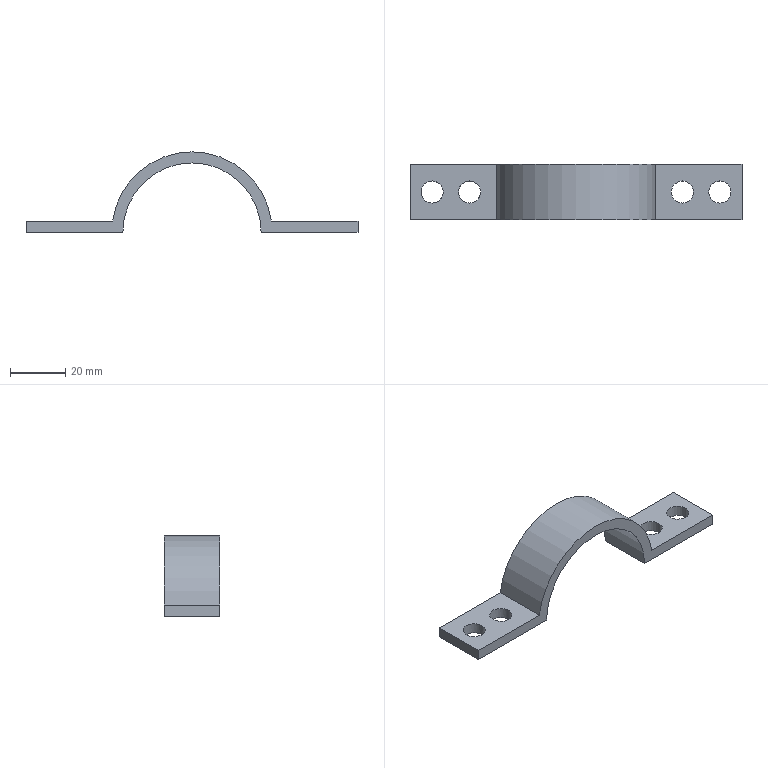Component | NX | TUTTTTUCU | 1 solid | 14 faces | volume 10956 mm3 | plane 8 | cylinder 6 | commonest cylinder face diameters 8 x4 58 x1 50 x1